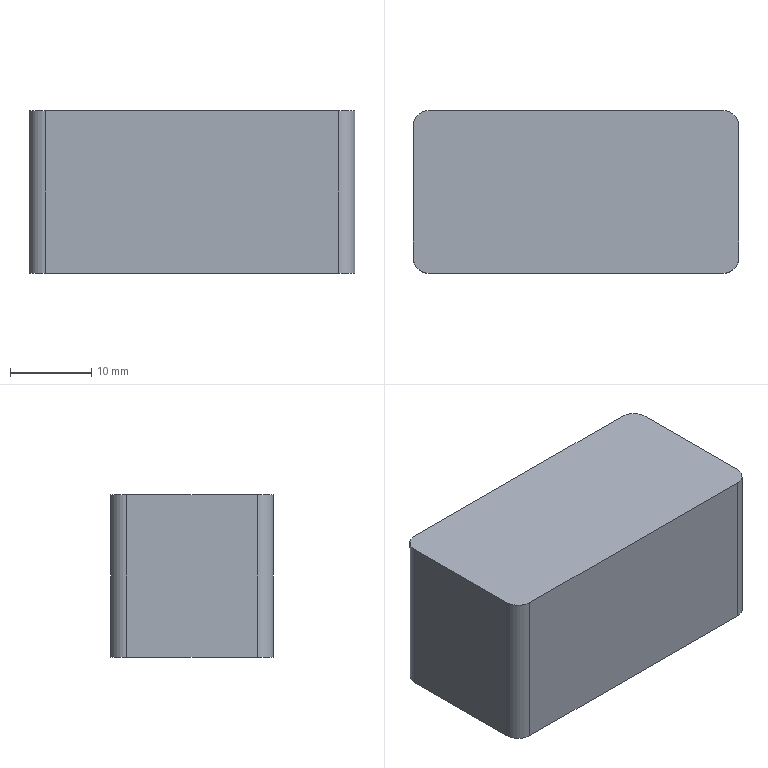Component | SolidWorks | WearBlock-1 | 1 solid | 10 faces | box 40 x 20 x 20 mm | volume 15931 mm3 | plane 6 | cylinder 4 | commonest cylinder face diameters 4 x4 | material H62
build123d program:
from build123d import *

# Parameters (mm, degrees)
BOSS_EXTRUDE1_DEPTH = 20


with BuildPart() as part:
    # Sketch1 → Boss-Extrude1 (new body)
    with BuildSketch(Plane.XY):
        with BuildLine():
            Line((18, -10), (-18, -10))
            ThreePointArc((-18, -10), (-19.414, -9.414), (-20, -8))
            Line((-20, -8), (-20, 8))
            ThreePointArc((-20, 8), (-19.414, 9.414), (-18, 10))
            Line((-18, 10), (18, 10))
            ThreePointArc((18, 10), (19.414, 9.414), (20, 8))
            Line((20, 8), (20, -8))
            ThreePointArc((20, -8), (19.414, -9.414), (18, -10))
        make_face()
    extrude(amount=BOSS_EXTRUDE1_DEPTH)


solid = part.part

# Placed as in the assembly
solid = solid.moved(Location((-179.87, -416.626, 692.215), (0, 0, 0)))
STEP:
#1=CARTESIAN_POINT('',(-6.294,-16.718,28.04));
#2=VERTEX_POINT('',#1);
#3=CARTESIAN_POINT('',(-6.373,-16.796,28.04));
#4=VERTEX_POINT('',#3);
#5=CARTESIAN_POINT('',(-6.373,-16.718,28.04));
#6=DIRECTION('',(0.,0.,-1.));
#7=DIRECTION('',(1.,0.,0.));
#8=AXIS2_PLACEMENT_3D('',#5,#6,#7);
#9=CIRCLE('',#8,0.07874);
#10=EDGE_CURVE('',#2,#4,#9,.T.);
#11=ORIENTED_EDGE('',*,*,#10,.T.);
#12=CARTESIAN_POINT('',(-6.373,-16.796,27.253));
#13=VERTEX_POINT('',#12);
#14=CARTESIAN_POINT('',(-6.373,-16.796,27.253));
#15=DIRECTION('',(-0.,-0.,1.));
#16=VECTOR('',#15,39.37);
#17=LINE('',#14,#16);
#18=EDGE_CURVE('',#13,#4,#17,.T.);
#19=ORIENTED_EDGE('',*,*,#18,.F.);
#20=CARTESIAN_POINT('',(-6.294,-16.718,27.253));
#21=VERTEX_POINT('',#20);
#22=CARTESIAN_POINT('',(-6.373,-16.718,27.253));
#23=DIRECTION('',(0.,0.,-1.));
#24=DIRECTION('',(1.,0.,0.));
#25=AXIS2_PLACEMENT_3D('',#22,#23,#24);
#26=CIRCLE('',#25,0.07874);
#27=EDGE_CURVE('',#21,#13,#26,.T.);
#28=ORIENTED_EDGE('',*,*,#27,.F.);
#29=CARTESIAN_POINT('',(-6.294,-16.718,27.253));
#30=DIRECTION('',(-0.,-0.,1.));
#31=VECTOR('',#30,39.37);
#32=LINE('',#29,#31);
#33=EDGE_CURVE('',#21,#2,#32,.T.);
#34=ORIENTED_EDGE('',*,*,#33,.T.);
#35=EDGE_LOOP('',(#11,#19,#28,#34));
#36=FACE_OUTER_BOUND('',#35,.T.);
#37=CARTESIAN_POINT('',(-6.373,-16.718,27.253));
#38=DIRECTION('',(-0.,-0.,1.));
#39=DIRECTION('',(1.,0.,0.));
#40=AXIS2_PLACEMENT_3D('',#37,#38,#39);
#41=CYLINDRICAL_SURFACE('',#40,0.07874);
#42=ADVANCED_FACE('',(#36),#41,.T.);
#43=CARTESIAN_POINT('',(-7.79,-16.796,28.04));
#44=VERTEX_POINT('',#43);
#45=CARTESIAN_POINT('',(-7.79,-16.796,28.04));
#46=DIRECTION('',(-1.,0.,-0.));
#47=VECTOR('',#46,39.37);
#48=LINE('',#45,#47);
#49=EDGE_CURVE('',#4,#44,#48,.T.);
#50=ORIENTED_EDGE('',*,*,#49,.T.);
#51=CARTESIAN_POINT('',(-7.79,-16.796,27.253));
#52=VERTEX_POINT('',#51);
#53=CARTESIAN_POINT('',(-7.79,-16.796,27.253));
#54=DIRECTION('',(-0.,-0.,1.));
#55=VECTOR('',#54,39.37);
#56=LINE('',#53,#55);
#57=EDGE_CURVE('',#52,#44,#56,.T.);
#58=ORIENTED_EDGE('',*,*,#57,.F.);
#59=CARTESIAN_POINT('',(-7.79,-16.796,27.253));
#60=DIRECTION('',(-1.,0.,-0.));
#61=VECTOR('',#60,39.37);
#62=LINE('',#59,#61);
#63=EDGE_CURVE('',#13,#52,#62,.T.);
#64=ORIENTED_EDGE('',*,*,#63,.F.);
#65=ORIENTED_EDGE('',*,*,#18,.T.);
#66=EDGE_LOOP('',(#50,#58,#64,#65));
#67=FACE_OUTER_BOUND('',#66,.T.);
#68=CARTESIAN_POINT('',(-7.79,-16.796,27.253));
#69=DIRECTION('',(0.,1.,0.));
#70=DIRECTION('',(0.,0.,-1.));
#71=AXIS2_PLACEMENT_3D('',#68,#69,#70);
#72=PLANE('',#71);
#73=ADVANCED_FACE('',(#67),#72,.F.);
#74=CARTESIAN_POINT('',(-7.869,-16.718,28.04));
#75=VERTEX_POINT('',#74);
#76=CARTESIAN_POINT('',(-7.79,-16.718,28.04));
#77=DIRECTION('',(0.,0.,-1.));
#78=DIRECTION('',(-1.,0.,0.));
#79=AXIS2_PLACEMENT_3D('',#76,#77,#78);
#80=CIRCLE('',#79,0.07874);
#81=EDGE_CURVE('',#44,#75,#80,.T.);
#82=ORIENTED_EDGE('',*,*,#81,.T.);
#83=CARTESIAN_POINT('',(-7.869,-16.718,27.253));
#84=VERTEX_POINT('',#83);
#85=CARTESIAN_POINT('',(-7.869,-16.718,27.253));
#86=DIRECTION('',(-0.,-0.,1.));
#87=VECTOR('',#86,39.37);
#88=LINE('',#85,#87);
#89=EDGE_CURVE('',#84,#75,#88,.T.);
#90=ORIENTED_EDGE('',*,*,#89,.F.);
#91=CARTESIAN_POINT('',(-7.79,-16.718,27.253));
#92=DIRECTION('',(0.,0.,-1.));
#93=DIRECTION('',(-1.,0.,0.));
#94=AXIS2_PLACEMENT_3D('',#91,#92,#93);
#95=CIRCLE('',#94,0.07874);
#96=EDGE_CURVE('',#52,#84,#95,.T.);
#97=ORIENTED_EDGE('',*,*,#96,.F.);
#98=ORIENTED_EDGE('',*,*,#57,.T.);
#99=EDGE_LOOP('',(#82,#90,#97,#98));
#100=FACE_OUTER_BOUND('',#99,.T.);
#101=CARTESIAN_POINT('',(-7.79,-16.718,27.253));
#102=DIRECTION('',(-0.,-0.,1.));
#103=DIRECTION('',(1.,0.,0.));
#104=AXIS2_PLACEMENT_3D('',#101,#102,#103);
#105=CYLINDRICAL_SURFACE('',#104,0.07874);
#106=ADVANCED_FACE('',(#100),#105,.T.);
#107=CARTESIAN_POINT('',(-7.869,-16.088,28.04));
#108=VERTEX_POINT('',#107);
#109=CARTESIAN_POINT('',(-7.869,-16.718,28.04));
#110=DIRECTION('',(0.,1.,0.));
#111=VECTOR('',#110,39.37);
#112=LINE('',#109,#111);
#113=EDGE_CURVE('',#75,#108,#112,.T.);
#114=ORIENTED_EDGE('',*,*,#113,.T.);
#115=CARTESIAN_POINT('',(-7.869,-16.088,27.253));
#116=VERTEX_POINT('',#115);
#117=CARTESIAN_POINT('',(-7.869,-16.088,27.253));
#118=DIRECTION('',(-0.,-0.,1.));
#119=VECTOR('',#118,39.37);
#120=LINE('',#117,#119);
#121=EDGE_CURVE('',#116,#108,#120,.T.);
#122=ORIENTED_EDGE('',*,*,#121,.F.);
#123=CARTESIAN_POINT('',(-7.869,-16.718,27.253));
#124=DIRECTION('',(0.,1.,0.));
#125=VECTOR('',#124,39.37);
#126=LINE('',#123,#125);
#127=EDGE_CURVE('',#84,#116,#126,.T.);
#128=ORIENTED_EDGE('',*,*,#127,.F.);
#129=ORIENTED_EDGE('',*,*,#89,.T.);
#130=EDGE_LOOP('',(#114,#122,#128,#129));
#131=FACE_OUTER_BOUND('',#130,.T.);
#132=CARTESIAN_POINT('',(-7.869,-16.718,27.253));
#133=DIRECTION('',(1.,-0.,0.));
#134=DIRECTION('',(0.,0.,-1.));
#135=AXIS2_PLACEMENT_3D('',#132,#133,#134);
#136=PLANE('',#135);
#137=ADVANCED_FACE('',(#131),#136,.F.);
#138=CARTESIAN_POINT('',(-7.79,-16.009,28.04));
#139=VERTEX_POINT('',#138);
#140=CARTESIAN_POINT('',(-7.79,-16.088,28.04));
#141=DIRECTION('',(0.,0.,-1.));
#142=DIRECTION('',(-1.,0.,0.));
#143=AXIS2_PLACEMENT_3D('',#140,#141,#142);
#144=CIRCLE('',#143,0.07874);
#145=EDGE_CURVE('',#108,#139,#144,.T.);
#146=ORIENTED_EDGE('',*,*,#145,.T.);
#147=CARTESIAN_POINT('',(-7.79,-16.009,27.253));
#148=VERTEX_POINT('',#147);
#149=CARTESIAN_POINT('',(-7.79,-16.009,27.253));
#150=DIRECTION('',(-0.,-0.,1.));
#151=VECTOR('',#150,39.37);
#152=LINE('',#149,#151);
#153=EDGE_CURVE('',#148,#139,#152,.T.);
#154=ORIENTED_EDGE('',*,*,#153,.F.);
#155=CARTESIAN_POINT('',(-7.79,-16.088,27.253));
#156=DIRECTION('',(0.,0.,-1.));
#157=DIRECTION('',(-1.,0.,0.));
#158=AXIS2_PLACEMENT_3D('',#155,#156,#157);
#159=CIRCLE('',#158,0.07874);
#160=EDGE_CURVE('',#116,#148,#159,.T.);
#161=ORIENTED_EDGE('',*,*,#160,.F.);
#162=ORIENTED_EDGE('',*,*,#121,.T.);
#163=EDGE_LOOP('',(#146,#154,#161,#162));
#164=FACE_OUTER_BOUND('',#163,.T.);
#165=CARTESIAN_POINT('',(-7.79,-16.088,27.253));
#166=DIRECTION('',(-0.,-0.,1.));
#167=DIRECTION('',(1.,0.,0.));
#168=AXIS2_PLACEMENT_3D('',#165,#166,#167);
#169=CYLINDRICAL_SURFACE('',#168,0.07874);
#170=ADVANCED_FACE('',(#164),#169,.T.);
#171=CARTESIAN_POINT('',(-6.373,-16.009,28.04));
#172=VERTEX_POINT('',#171);
#173=CARTESIAN_POINT('',(-7.79,-16.009,28.04));
#174=DIRECTION('',(1.,-0.,0.));
#175=VECTOR('',#174,39.37);
#176=LINE('',#173,#175);
#177=EDGE_CURVE('',#139,#172,#176,.T.);
#178=ORIENTED_EDGE('',*,*,#177,.T.);
#179=CARTESIAN_POINT('',(-6.373,-16.009,27.253));
#180=VERTEX_POINT('',#179);
#181=CARTESIAN_POINT('',(-6.373,-16.009,27.253));
#182=DIRECTION('',(-0.,-0.,1.));
#183=VECTOR('',#182,39.37);
#184=LINE('',#181,#183);
#185=EDGE_CURVE('',#180,#172,#184,.T.);
#186=ORIENTED_EDGE('',*,*,#185,.F.);
#187=CARTESIAN_POINT('',(-7.79,-16.009,27.253));
#188=DIRECTION('',(1.,-0.,0.));
#189=VECTOR('',#188,39.37);
#190=LINE('',#187,#189);
#191=EDGE_CURVE('',#148,#180,#190,.T.);
#192=ORIENTED_EDGE('',*,*,#191,.F.);
#193=ORIENTED_EDGE('',*,*,#153,.T.);
#194=EDGE_LOOP('',(#178,#186,#192,#193));
#195=FACE_OUTER_BOUND('',#194,.T.);
#196=CARTESIAN_POINT('',(-7.79,-16.009,27.253));
#197=DIRECTION('',(-0.,-1.,-0.));
#198=DIRECTION('',(-1.,0.,-0.));
#199=AXIS2_PLACEMENT_3D('',#196,#197,#198);
#200=PLANE('',#199);
#201=ADVANCED_FACE('',(#195),#200,.F.);
#202=CARTESIAN_POINT('',(-6.294,-16.088,28.04));
#203=VERTEX_POINT('',#202);
#204=CARTESIAN_POINT('',(-6.373,-16.088,28.04));
#205=DIRECTION('',(0.,0.,-1.));
#206=DIRECTION('',(-1.,0.,0.));
#207=AXIS2_PLACEMENT_3D('',#204,#205,#206);
#208=CIRCLE('',#207,0.07874);
#209=EDGE_CURVE('',#172,#203,#208,.T.);
#210=ORIENTED_EDGE('',*,*,#209,.T.);
#211=CARTESIAN_POINT('',(-6.294,-16.088,27.253));
#212=VERTEX_POINT('',#211);
#213=CARTESIAN_POINT('',(-6.294,-16.088,27.253));
#214=DIRECTION('',(-0.,-0.,1.));
#215=VECTOR('',#214,39.37);
#216=LINE('',#213,#215);
#217=EDGE_CURVE('',#212,#203,#216,.T.);
#218=ORIENTED_EDGE('',*,*,#217,.F.);
#219=CARTESIAN_POINT('',(-6.373,-16.088,27.253));
#220=DIRECTION('',(0.,0.,-1.));
#221=DIRECTION('',(-1.,0.,0.));
#222=AXIS2_PLACEMENT_3D('',#219,#220,#221);
#223=CIRCLE('',#222,0.07874);
#224=EDGE_CURVE('',#180,#212,#223,.T.);
#225=ORIENTED_EDGE('',*,*,#224,.F.);
#226=ORIENTED_EDGE('',*,*,#185,.T.);
#227=EDGE_LOOP('',(#210,#218,#225,#226));
#228=FACE_OUTER_BOUND('',#227,.T.);
#229=CARTESIAN_POINT('',(-6.373,-16.088,27.253));
#230=DIRECTION('',(-0.,-0.,1.));
#231=DIRECTION('',(1.,0.,0.));
#232=AXIS2_PLACEMENT_3D('',#229,#230,#231);
#233=CYLINDRICAL_SURFACE('',#232,0.07874);
#234=ADVANCED_FACE('',(#228),#233,.T.);
#235=CARTESIAN_POINT('',(-6.294,-16.718,28.04));
#236=DIRECTION('',(-0.,-1.,-0.));
#237=VECTOR('',#236,39.37);
#238=LINE('',#235,#237);
#239=EDGE_CURVE('',#203,#2,#238,.T.);
#240=ORIENTED_EDGE('',*,*,#239,.T.);
#241=ORIENTED_EDGE('',*,*,#33,.F.);
#242=CARTESIAN_POINT('',(-6.294,-16.718,27.253));
#243=DIRECTION('',(-0.,-1.,-0.));
#244=VECTOR('',#243,39.37);
#245=LINE('',#242,#244);
#246=EDGE_CURVE('',#212,#21,#245,.T.);
#247=ORIENTED_EDGE('',*,*,#246,.F.);
#248=ORIENTED_EDGE('',*,*,#217,.T.);
#249=EDGE_LOOP('',(#240,#241,#247,#248));
#250=FACE_OUTER_BOUND('',#249,.T.);
#251=CARTESIAN_POINT('',(-6.294,-16.718,27.253));
#252=DIRECTION('',(-1.,0.,-0.));
#253=DIRECTION('',(-0.,-0.,1.));
#254=AXIS2_PLACEMENT_3D('',#251,#252,#253);
#255=PLANE('',#254);
#256=ADVANCED_FACE('',(#250),#255,.F.);
#257=ORIENTED_EDGE('',*,*,#27,.T.);
#258=ORIENTED_EDGE('',*,*,#63,.T.);
#259=ORIENTED_EDGE('',*,*,#96,.T.);
#260=ORIENTED_EDGE('',*,*,#127,.T.);
#261=ORIENTED_EDGE('',*,*,#160,.T.);
#262=ORIENTED_EDGE('',*,*,#191,.T.);
#263=ORIENTED_EDGE('',*,*,#224,.T.);
#264=ORIENTED_EDGE('',*,*,#246,.T.);
#265=EDGE_LOOP('',(#257,#258,#259,#260,#261,#262,#263,#264));
#266=FACE_OUTER_BOUND('',#265,.T.);
#267=CARTESIAN_POINT('',(-6.373,-16.718,27.253));
#268=DIRECTION('',(-0.,-0.,1.));
#269=DIRECTION('',(1.,-0.,0.));
#270=AXIS2_PLACEMENT_3D('',#267,#268,#269);
#271=PLANE('',#270);
#272=ADVANCED_FACE('',(#266),#271,.F.);
#273=ORIENTED_EDGE('',*,*,#10,.F.);
#274=ORIENTED_EDGE('',*,*,#239,.F.);
#275=ORIENTED_EDGE('',*,*,#209,.F.);
#276=ORIENTED_EDGE('',*,*,#177,.F.);
#277=ORIENTED_EDGE('',*,*,#145,.F.);
#278=ORIENTED_EDGE('',*,*,#113,.F.);
#279=ORIENTED_EDGE('',*,*,#81,.F.);
#280=ORIENTED_EDGE('',*,*,#49,.F.);
#281=EDGE_LOOP('',(#273,#274,#275,#276,#277,#278,#279,#280));
#282=FACE_OUTER_BOUND('',#281,.T.);
#283=CARTESIAN_POINT('',(-6.373,-16.718,28.04));
#284=DIRECTION('',(-0.,-0.,1.));
#285=DIRECTION('',(1.,-0.,0.));
#286=AXIS2_PLACEMENT_3D('',#283,#284,#285);
#287=PLANE('',#286);
#288=ADVANCED_FACE('',(#282),#287,.T.);
#289=CLOSED_SHELL('',(#42,#73,#106,#137,#170,#201,#234,#256,#272,#288));
#290=MANIFOLD_SOLID_BREP('',#289);
#291=CARTESIAN_POINT('',(0.,0.,0.));
#292=DIRECTION('',(0.,0.,1.));
#293=DIRECTION('',(1.,0.,0.));
#294=AXIS2_PLACEMENT_3D('',#291,#292,#293);
#295=(LENGTH_UNIT()NAMED_UNIT(*)SI_UNIT($,.METRE.));
#296=LENGTH_MEASURE_WITH_UNIT(LENGTH_MEASURE(0.0254),#295);
#297=DIMENSIONAL_EXPONENTS(1.,0.,0.,0.,0.,0.,0.);
#298=(CONVERSION_BASED_UNIT('',#296)LENGTH_UNIT()NAMED_UNIT(#297));
#299=UNCERTAINTY_MEASURE_WITH_UNIT(LENGTH_MEASURE(0.00001),#298,'','');
#300=(NAMED_UNIT(*)PLANE_ANGLE_UNIT()SI_UNIT($,.RADIAN.));
#301=(NAMED_UNIT(*)SI_UNIT($,.STERADIAN.)SOLID_ANGLE_UNIT());
#302=(GEOMETRIC_REPRESENTATION_CONTEXT(3)GLOBAL_UNCERTAINTY_ASSIGNED_CONTEXT((#299))GLOBAL_UNIT_ASSIGNED_CONTEXT((#298,#300,#301))REPRESENTATION_CONTEXT('',''));
#303=ADVANCED_BREP_SHAPE_REPRESENTATION('',(#290,#294),#302);
#304=COLOUR_RGB('',0.7922,0.8196,0.9333);
#305=FILL_AREA_STYLE_COLOUR('',#304);
#306=FILL_AREA_STYLE('',(#305));
#307=SURFACE_STYLE_FILL_AREA(#306);
#308=SURFACE_SIDE_STYLE('',(#307));
#309=SURFACE_STYLE_USAGE(.BOTH.,#308);
#310=PRESENTATION_STYLE_ASSIGNMENT((#309));
#311=STYLED_ITEM('',(#310),#290);
#312=(LENGTH_UNIT()NAMED_UNIT(*)SI_UNIT($,.METRE.));
#313=LENGTH_MEASURE_WITH_UNIT(LENGTH_MEASURE(0.0254),#312);
#314=DIMENSIONAL_EXPONENTS(1.,0.,0.,0.,0.,0.,0.);
#315=(CONVERSION_BASED_UNIT('',#313)LENGTH_UNIT()NAMED_UNIT(#314));
#316=UNCERTAINTY_MEASURE_WITH_UNIT(LENGTH_MEASURE(0.00001),#315,'','');
#317=(NAMED_UNIT(*)PLANE_ANGLE_UNIT()SI_UNIT($,.RADIAN.));
#318=(NAMED_UNIT(*)SI_UNIT($,.STERADIAN.)SOLID_ANGLE_UNIT());
#319=(GEOMETRIC_REPRESENTATION_CONTEXT(3)GLOBAL_UNCERTAINTY_ASSIGNED_CONTEXT((#316))GLOBAL_UNIT_ASSIGNED_CONTEXT((#315,#317,#318))REPRESENTATION_CONTEXT('',''));
#320=MECHANICAL_DESIGN_GEOMETRIC_PRESENTATION_REPRESENTATION('',(#311),#319);
#321=PRESENTATION_LAYER_ASSIGNMENT('','',(#311));